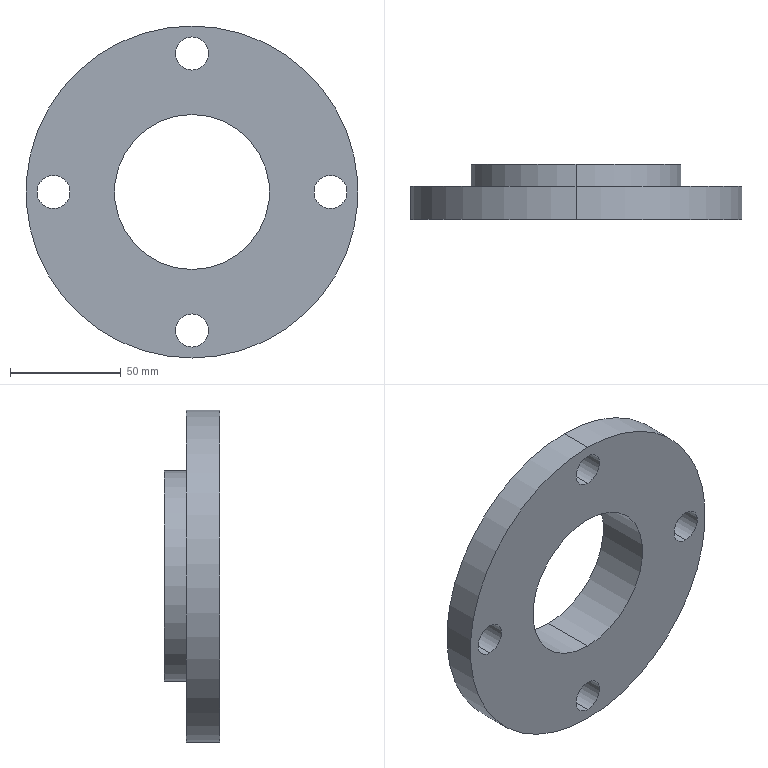Component | SolidWorks | SupportLeg-2 | 1 solid | 17 faces | box 150 x 25 x 150 mm | volume 229140 mm3 | cylinder 14 | plane 3 | commonest cylinder face diameters 15 x8 95 x2 70 x2 150 x2
build123d program:
from build123d import *

# Parameters (mm, degrees)
SKETCH1_R           = 75
SKETCH1_R_2         = 35
SKETCH1_R_3         = 7.5
BOSS_EXTRUDE1_DEPTH = 15
SKETCH2_R           = 47.5
SKETCH2_R_2         = 35
BOSS_EXTRUDE2_DEPTH = 10


with BuildPart() as part:
    # Sketch1 → Boss-Extrude1 (new body)
    with BuildSketch(Plane(origin=(0, 0, 0), x_dir=(1, 0, 0), z_dir=(0, 1, 0))):
        with Locations(Location((0, 0, 0), (0, 0, 270))):
            Circle(SKETCH1_R)
        with Locations(Location((0, 0, 0), (0, 0, 270))):
            Circle(SKETCH1_R_2, mode=Mode.SUBTRACT)
        with Locations(Location((0, 62.566, 0), (0, 0, 270))):
            Circle(SKETCH1_R_3, mode=Mode.SUBTRACT)
        with Locations(Location((62.566, 0, 0), (0, 0, 270))):
            Circle(SKETCH1_R_3, mode=Mode.SUBTRACT)
        with Locations(Location((0, -62.566, 0), (0, 0, 270))):
            Circle(SKETCH1_R_3, mode=Mode.SUBTRACT)
        with Locations(Location((-62.566, 0, 0), (0, 0, 270))):
            Circle(SKETCH1_R_3, mode=Mode.SUBTRACT)
    extrude(amount=BOSS_EXTRUDE1_DEPTH)

    # Sketch2 → Boss-Extrude2 (add)
    with BuildSketch(Plane(origin=(0, 15, 0), x_dir=(1, 0, 0), z_dir=(0, 1, 0))):
        with Locations(Location((0, 0, 0), (0, 0, 270))):
            Circle(SKETCH2_R)
        with Locations(Location((0, 0, 0), (0, 0, 270))):
            Circle(SKETCH2_R_2, mode=Mode.SUBTRACT)
    extrude(amount=BOSS_EXTRUDE2_DEPTH)


solid = part.part

# Placed as in the assembly
solid = solid.moved(Location((-699.263, -180, 149.263), (0, 0, 0)))
STEP:
#1=COLOUR_RGB('',0.7922,0.8196,0.9333);
#2=FILL_AREA_STYLE_COLOUR('',#1);
#3=FILL_AREA_STYLE('',(#2));
#4=SURFACE_STYLE_FILL_AREA(#3);
#5=SURFACE_SIDE_STYLE('',(#4));
#6=SURFACE_STYLE_USAGE(.BOTH.,#5);
#7=PRESENTATION_STYLE_ASSIGNMENT((#6));
#8=CARTESIAN_POINT('',(-27.53,-6.102,7.747));
#9=VERTEX_POINT('',#8);
#10=CARTESIAN_POINT('',(-27.53,-6.102,4.006));
#11=VERTEX_POINT('',#10);
#12=CARTESIAN_POINT('',(-27.53,-6.102,5.877));
#13=DIRECTION('',(0.,1.,0.));
#14=DIRECTION('',(0.,0.,1.));
#15=AXIS2_PLACEMENT_3D('',#12,#13,#14);
#16=CIRCLE('',#15,1.87);
#17=EDGE_CURVE('',#9,#11,#16,.T.);
#18=ORIENTED_EDGE('',*,*,#17,.F.);
#19=CARTESIAN_POINT('',(-27.53,-6.496,7.747));
#20=VERTEX_POINT('',#19);
#21=CARTESIAN_POINT('',(-27.53,-6.102,7.747));
#22=DIRECTION('',(0.,-1.,0.));
#23=VECTOR('',#22,39.37);
#24=LINE('',#21,#23);
#25=EDGE_CURVE('',#9,#20,#24,.T.);
#26=ORIENTED_EDGE('',*,*,#25,.T.);
#27=CARTESIAN_POINT('',(-27.53,-6.496,4.006));
#28=VERTEX_POINT('',#27);
#29=CARTESIAN_POINT('',(-27.53,-6.496,5.877));
#30=DIRECTION('',(0.,1.,0.));
#31=DIRECTION('',(0.,0.,1.));
#32=AXIS2_PLACEMENT_3D('',#29,#30,#31);
#33=CIRCLE('',#32,1.87);
#34=EDGE_CURVE('',#20,#28,#33,.T.);
#35=ORIENTED_EDGE('',*,*,#34,.T.);
#36=CARTESIAN_POINT('',(-27.53,-6.102,4.006));
#37=DIRECTION('',(0.,-1.,0.));
#38=VECTOR('',#37,39.37);
#39=LINE('',#36,#38);
#40=EDGE_CURVE('',#11,#28,#39,.T.);
#41=ORIENTED_EDGE('',*,*,#40,.F.);
#42=EDGE_LOOP('',(#18,#26,#35,#41));
#43=FACE_OUTER_BOUND('',#42,.T.);
#44=CARTESIAN_POINT('',(-27.53,-6.102,5.877));
#45=DIRECTION('',(0.,-1.,0.));
#46=DIRECTION('',(0.,0.,-1.));
#47=AXIS2_PLACEMENT_3D('',#44,#45,#46);
#48=CYLINDRICAL_SURFACE('',#47,1.87);
#49=ADVANCED_FACE('',(#43),#48,.T.);
#50=CARTESIAN_POINT('',(-29.993,-6.496,5.581));
#51=VERTEX_POINT('',#50);
#52=CARTESIAN_POINT('',(-29.993,-6.496,6.172));
#53=VERTEX_POINT('',#52);
#54=CARTESIAN_POINT('',(-29.993,-6.496,5.877));
#55=DIRECTION('',(0.,1.,0.));
#56=DIRECTION('',(0.,0.,1.));
#57=AXIS2_PLACEMENT_3D('',#54,#55,#56);
#58=CIRCLE('',#57,0.2953);
#59=EDGE_CURVE('',#51,#53,#58,.T.);
#60=ORIENTED_EDGE('',*,*,#59,.T.);
#61=CARTESIAN_POINT('',(-29.993,-7.087,6.172));
#62=VERTEX_POINT('',#61);
#63=CARTESIAN_POINT('',(-29.993,-6.496,6.172));
#64=DIRECTION('',(0.,-1.,0.));
#65=VECTOR('',#64,39.37);
#66=LINE('',#63,#65);
#67=EDGE_CURVE('',#53,#62,#66,.T.);
#68=ORIENTED_EDGE('',*,*,#67,.T.);
#69=CARTESIAN_POINT('',(-29.993,-7.087,5.581));
#70=VERTEX_POINT('',#69);
#71=CARTESIAN_POINT('',(-29.993,-7.087,5.877));
#72=DIRECTION('',(0.,1.,0.));
#73=DIRECTION('',(0.,0.,1.));
#74=AXIS2_PLACEMENT_3D('',#71,#72,#73);
#75=CIRCLE('',#74,0.2953);
#76=EDGE_CURVE('',#70,#62,#75,.T.);
#77=ORIENTED_EDGE('',*,*,#76,.F.);
#78=CARTESIAN_POINT('',(-29.993,-6.496,5.581));
#79=DIRECTION('',(0.,-1.,0.));
#80=VECTOR('',#79,39.37);
#81=LINE('',#78,#80);
#82=EDGE_CURVE('',#51,#70,#81,.T.);
#83=ORIENTED_EDGE('',*,*,#82,.F.);
#84=EDGE_LOOP('',(#60,#68,#77,#83));
#85=FACE_OUTER_BOUND('',#84,.T.);
#86=CARTESIAN_POINT('',(-29.993,-6.496,5.877));
#87=DIRECTION('',(0.,-1.,0.));
#88=DIRECTION('',(0.,0.,-1.));
#89=AXIS2_PLACEMENT_3D('',#86,#87,#88);
#90=CYLINDRICAL_SURFACE('',#89,0.2953);
#91=ADVANCED_FACE('',(#85),#90,.F.);
#92=CARTESIAN_POINT('',(-27.53,-6.496,8.044));
#93=VERTEX_POINT('',#92);
#94=CARTESIAN_POINT('',(-27.53,-6.496,8.635));
#95=VERTEX_POINT('',#94);
#96=CARTESIAN_POINT('',(-27.53,-6.496,8.34));
#97=DIRECTION('',(0.,1.,0.));
#98=DIRECTION('',(0.,0.,1.));
#99=AXIS2_PLACEMENT_3D('',#96,#97,#98);
#100=CIRCLE('',#99,0.2953);
#101=EDGE_CURVE('',#93,#95,#100,.T.);
#102=ORIENTED_EDGE('',*,*,#101,.T.);
#103=CARTESIAN_POINT('',(-27.53,-7.087,8.635));
#104=VERTEX_POINT('',#103);
#105=CARTESIAN_POINT('',(-27.53,-6.496,8.635));
#106=DIRECTION('',(0.,-1.,0.));
#107=VECTOR('',#106,39.37);
#108=LINE('',#105,#107);
#109=EDGE_CURVE('',#95,#104,#108,.T.);
#110=ORIENTED_EDGE('',*,*,#109,.T.);
#111=CARTESIAN_POINT('',(-27.53,-7.087,8.044));
#112=VERTEX_POINT('',#111);
#113=CARTESIAN_POINT('',(-27.53,-7.087,8.34));
#114=DIRECTION('',(0.,1.,0.));
#115=DIRECTION('',(0.,0.,1.));
#116=AXIS2_PLACEMENT_3D('',#113,#114,#115);
#117=CIRCLE('',#116,0.2953);
#118=EDGE_CURVE('',#112,#104,#117,.T.);
#119=ORIENTED_EDGE('',*,*,#118,.F.);
#120=CARTESIAN_POINT('',(-27.53,-6.496,8.044));
#121=DIRECTION('',(0.,-1.,0.));
#122=VECTOR('',#121,39.37);
#123=LINE('',#120,#122);
#124=EDGE_CURVE('',#93,#112,#123,.T.);
#125=ORIENTED_EDGE('',*,*,#124,.F.);
#126=EDGE_LOOP('',(#102,#110,#119,#125));
#127=FACE_OUTER_BOUND('',#126,.T.);
#128=CARTESIAN_POINT('',(-27.53,-6.496,8.34));
#129=DIRECTION('',(0.,-1.,0.));
#130=DIRECTION('',(0.,0.,-1.));
#131=AXIS2_PLACEMENT_3D('',#128,#129,#130);
#132=CYLINDRICAL_SURFACE('',#131,0.2953);
#133=ADVANCED_FACE('',(#127),#132,.F.);
#134=CARTESIAN_POINT('',(-25.067,-6.496,5.581));
#135=VERTEX_POINT('',#134);
#136=CARTESIAN_POINT('',(-25.067,-6.496,6.172));
#137=VERTEX_POINT('',#136);
#138=CARTESIAN_POINT('',(-25.067,-6.496,5.877));
#139=DIRECTION('',(0.,1.,0.));
#140=DIRECTION('',(0.,0.,1.));
#141=AXIS2_PLACEMENT_3D('',#138,#139,#140);
#142=CIRCLE('',#141,0.2953);
#143=EDGE_CURVE('',#135,#137,#142,.T.);
#144=ORIENTED_EDGE('',*,*,#143,.T.);
#145=CARTESIAN_POINT('',(-25.067,-7.087,6.172));
#146=VERTEX_POINT('',#145);
#147=CARTESIAN_POINT('',(-25.067,-6.496,6.172));
#148=DIRECTION('',(0.,-1.,0.));
#149=VECTOR('',#148,39.37);
#150=LINE('',#147,#149);
#151=EDGE_CURVE('',#137,#146,#150,.T.);
#152=ORIENTED_EDGE('',*,*,#151,.T.);
#153=CARTESIAN_POINT('',(-25.067,-7.087,5.581));
#154=VERTEX_POINT('',#153);
#155=CARTESIAN_POINT('',(-25.067,-7.087,5.877));
#156=DIRECTION('',(0.,1.,0.));
#157=DIRECTION('',(0.,0.,1.));
#158=AXIS2_PLACEMENT_3D('',#155,#156,#157);
#159=CIRCLE('',#158,0.2953);
#160=EDGE_CURVE('',#154,#146,#159,.T.);
#161=ORIENTED_EDGE('',*,*,#160,.F.);
#162=CARTESIAN_POINT('',(-25.067,-6.496,5.581));
#163=DIRECTION('',(0.,-1.,0.));
#164=VECTOR('',#163,39.37);
#165=LINE('',#162,#164);
#166=EDGE_CURVE('',#135,#154,#165,.T.);
#167=ORIENTED_EDGE('',*,*,#166,.F.);
#168=EDGE_LOOP('',(#144,#152,#161,#167));
#169=FACE_OUTER_BOUND('',#168,.T.);
#170=CARTESIAN_POINT('',(-25.067,-6.496,5.877));
#171=DIRECTION('',(0.,-1.,0.));
#172=DIRECTION('',(0.,0.,-1.));
#173=AXIS2_PLACEMENT_3D('',#170,#171,#172);
#174=CYLINDRICAL_SURFACE('',#173,0.2953);
#175=ADVANCED_FACE('',(#169),#174,.F.);
#176=CARTESIAN_POINT('',(-27.53,-6.496,3.118));
#177=VERTEX_POINT('',#176);
#178=CARTESIAN_POINT('',(-27.53,-6.496,3.709));
#179=VERTEX_POINT('',#178);
#180=CARTESIAN_POINT('',(-27.53,-6.496,3.413));
#181=DIRECTION('',(0.,1.,0.));
#182=DIRECTION('',(0.,0.,1.));
#183=AXIS2_PLACEMENT_3D('',#180,#181,#182);
#184=CIRCLE('',#183,0.2953);
#185=EDGE_CURVE('',#177,#179,#184,.T.);
#186=ORIENTED_EDGE('',*,*,#185,.T.);
#187=CARTESIAN_POINT('',(-27.53,-7.087,3.709));
#188=VERTEX_POINT('',#187);
#189=CARTESIAN_POINT('',(-27.53,-6.496,3.709));
#190=DIRECTION('',(0.,-1.,0.));
#191=VECTOR('',#190,39.37);
#192=LINE('',#189,#191);
#193=EDGE_CURVE('',#179,#188,#192,.T.);
#194=ORIENTED_EDGE('',*,*,#193,.T.);
#195=CARTESIAN_POINT('',(-27.53,-7.087,3.118));
#196=VERTEX_POINT('',#195);
#197=CARTESIAN_POINT('',(-27.53,-7.087,3.413));
#198=DIRECTION('',(0.,1.,0.));
#199=DIRECTION('',(0.,0.,1.));
#200=AXIS2_PLACEMENT_3D('',#197,#198,#199);
#201=CIRCLE('',#200,0.2953);
#202=EDGE_CURVE('',#196,#188,#201,.T.);
#203=ORIENTED_EDGE('',*,*,#202,.F.);
#204=CARTESIAN_POINT('',(-27.53,-6.496,3.118));
#205=DIRECTION('',(0.,-1.,0.));
#206=VECTOR('',#205,39.37);
#207=LINE('',#204,#206);
#208=EDGE_CURVE('',#177,#196,#207,.T.);
#209=ORIENTED_EDGE('',*,*,#208,.F.);
#210=EDGE_LOOP('',(#186,#194,#203,#209));
#211=FACE_OUTER_BOUND('',#210,.T.);
#212=CARTESIAN_POINT('',(-27.53,-6.496,3.413));
#213=DIRECTION('',(0.,-1.,0.));
#214=DIRECTION('',(0.,0.,-1.));
#215=AXIS2_PLACEMENT_3D('',#212,#213,#214);
#216=CYLINDRICAL_SURFACE('',#215,0.2953);
#217=ADVANCED_FACE('',(#211),#216,.F.);
#218=CARTESIAN_POINT('',(-27.53,-6.102,4.499));
#219=VERTEX_POINT('',#218);
#220=CARTESIAN_POINT('',(-27.53,-6.102,7.254));
#221=VERTEX_POINT('',#220);
#222=CARTESIAN_POINT('',(-27.53,-6.102,5.877));
#223=DIRECTION('',(0.,1.,0.));
#224=DIRECTION('',(0.,0.,1.));
#225=AXIS2_PLACEMENT_3D('',#222,#223,#224);
#226=CIRCLE('',#225,1.378);
#227=EDGE_CURVE('',#219,#221,#226,.T.);
#228=ORIENTED_EDGE('',*,*,#227,.T.);
#229=CARTESIAN_POINT('',(-27.53,-7.087,7.254));
#230=VERTEX_POINT('',#229);
#231=CARTESIAN_POINT('',(-27.53,-6.496,7.254));
#232=DIRECTION('',(0.,-1.,0.));
#233=VECTOR('',#232,39.37);
#234=LINE('',#231,#233);
#235=EDGE_CURVE('',#221,#230,#234,.T.);
#236=ORIENTED_EDGE('',*,*,#235,.T.);
#237=CARTESIAN_POINT('',(-27.53,-7.087,4.499));
#238=VERTEX_POINT('',#237);
#239=CARTESIAN_POINT('',(-27.53,-7.087,5.877));
#240=DIRECTION('',(0.,1.,0.));
#241=DIRECTION('',(0.,0.,1.));
#242=AXIS2_PLACEMENT_3D('',#239,#240,#241);
#243=CIRCLE('',#242,1.378);
#244=EDGE_CURVE('',#238,#230,#243,.T.);
#245=ORIENTED_EDGE('',*,*,#244,.F.);
#246=CARTESIAN_POINT('',(-27.53,-6.496,4.499));
#247=DIRECTION('',(0.,-1.,0.));
#248=VECTOR('',#247,39.37);
#249=LINE('',#246,#248);
#250=EDGE_CURVE('',#219,#238,#249,.T.);
#251=ORIENTED_EDGE('',*,*,#250,.F.);
#252=EDGE_LOOP('',(#228,#236,#245,#251));
#253=FACE_OUTER_BOUND('',#252,.T.);
#254=CARTESIAN_POINT('',(-27.53,-6.496,5.877));
#255=DIRECTION('',(0.,-1.,0.));
#256=DIRECTION('',(0.,0.,-1.));
#257=AXIS2_PLACEMENT_3D('',#254,#255,#256);
#258=CYLINDRICAL_SURFACE('',#257,1.378);
#259=ADVANCED_FACE('',(#253),#258,.F.);
#260=CARTESIAN_POINT('',(-27.53,-6.496,8.829));
#261=VERTEX_POINT('',#260);
#262=CARTESIAN_POINT('',(-27.53,-6.496,2.924));
#263=VERTEX_POINT('',#262);
#264=CARTESIAN_POINT('',(-27.53,-6.496,5.877));
#265=DIRECTION('',(0.,1.,0.));
#266=DIRECTION('',(0.,0.,1.));
#267=AXIS2_PLACEMENT_3D('',#264,#265,#266);
#268=CIRCLE('',#267,2.953);
#269=EDGE_CURVE('',#261,#263,#268,.T.);
#270=ORIENTED_EDGE('',*,*,#269,.F.);
#271=CARTESIAN_POINT('',(-27.53,-7.087,8.829));
#272=VERTEX_POINT('',#271);
#273=CARTESIAN_POINT('',(-27.53,-6.496,8.829));
#274=DIRECTION('',(0.,-1.,0.));
#275=VECTOR('',#274,39.37);
#276=LINE('',#273,#275);
#277=EDGE_CURVE('',#261,#272,#276,.T.);
#278=ORIENTED_EDGE('',*,*,#277,.T.);
#279=CARTESIAN_POINT('',(-27.53,-7.087,2.924));
#280=VERTEX_POINT('',#279);
#281=CARTESIAN_POINT('',(-27.53,-7.087,5.877));
#282=DIRECTION('',(0.,1.,0.));
#283=DIRECTION('',(0.,0.,1.));
#284=AXIS2_PLACEMENT_3D('',#281,#282,#283);
#285=CIRCLE('',#284,2.953);
#286=EDGE_CURVE('',#272,#280,#285,.T.);
#287=ORIENTED_EDGE('',*,*,#286,.T.);
#288=CARTESIAN_POINT('',(-27.53,-6.496,2.924));
#289=DIRECTION('',(0.,-1.,0.));
#290=VECTOR('',#289,39.37);
#291=LINE('',#288,#290);
#292=EDGE_CURVE('',#263,#280,#291,.T.);
#293=ORIENTED_EDGE('',*,*,#292,.F.);
#294=EDGE_LOOP('',(#270,#278,#287,#293));
#295=FACE_OUTER_BOUND('',#294,.T.);
#296=CARTESIAN_POINT('',(-27.53,-6.496,5.877));
#297=DIRECTION('',(0.,-1.,0.));
#298=DIRECTION('',(0.,0.,-1.));
#299=AXIS2_PLACEMENT_3D('',#296,#297,#298);
#300=CYLINDRICAL_SURFACE('',#299,2.953);
#301=ADVANCED_FACE('',(#295),#300,.T.);
#302=CARTESIAN_POINT('',(-27.53,-6.496,5.877));
#303=DIRECTION('',(0.,1.,0.));
#304=DIRECTION('',(0.,0.,1.));
#305=AXIS2_PLACEMENT_3D('',#302,#303,#304);
#306=CIRCLE('',#305,1.87);
#307=EDGE_CURVE('',#28,#20,#306,.T.);
#308=ORIENTED_EDGE('',*,*,#307,.F.);
#309=ORIENTED_EDGE('',*,*,#34,.F.);
#310=EDGE_LOOP('',(#308,#309));
#311=FACE_BOUND('',#310,.T.);
#312=ORIENTED_EDGE('',*,*,#101,.F.);
#313=CARTESIAN_POINT('',(-27.53,-6.496,8.34));
#314=DIRECTION('',(0.,1.,0.));
#315=DIRECTION('',(0.,0.,1.));
#316=AXIS2_PLACEMENT_3D('',#313,#314,#315);
#317=CIRCLE('',#316,0.2953);
#318=EDGE_CURVE('',#95,#93,#317,.T.);
#319=ORIENTED_EDGE('',*,*,#318,.F.);
#320=EDGE_LOOP('',(#312,#319));
#321=FACE_BOUND('',#320,.T.);
#322=ORIENTED_EDGE('',*,*,#185,.F.);
#323=CARTESIAN_POINT('',(-27.53,-6.496,3.413));
#324=DIRECTION('',(0.,1.,0.));
#325=DIRECTION('',(0.,0.,1.));
#326=AXIS2_PLACEMENT_3D('',#323,#324,#325);
#327=CIRCLE('',#326,0.2953);
#328=EDGE_CURVE('',#179,#177,#327,.T.);
#329=ORIENTED_EDGE('',*,*,#328,.F.);
#330=EDGE_LOOP('',(#322,#329));
#331=FACE_BOUND('',#330,.T.);
#332=CARTESIAN_POINT('',(-27.53,-6.496,5.877));
#333=DIRECTION('',(0.,1.,0.));
#334=DIRECTION('',(0.,0.,1.));
#335=AXIS2_PLACEMENT_3D('',#332,#333,#334);
#336=CIRCLE('',#335,2.953);
#337=EDGE_CURVE('',#263,#261,#336,.T.);
#338=ORIENTED_EDGE('',*,*,#337,.T.);
#339=ORIENTED_EDGE('',*,*,#269,.T.);
#340=EDGE_LOOP('',(#338,#339));
#341=FACE_OUTER_BOUND('',#340,.T.);
#342=ORIENTED_EDGE('',*,*,#143,.F.);
#343=CARTESIAN_POINT('',(-25.067,-6.496,5.877));
#344=DIRECTION('',(0.,1.,0.));
#345=DIRECTION('',(0.,0.,1.));
#346=AXIS2_PLACEMENT_3D('',#343,#344,#345);
#347=CIRCLE('',#346,0.2953);
#348=EDGE_CURVE('',#137,#135,#347,.T.);
#349=ORIENTED_EDGE('',*,*,#348,.F.);
#350=EDGE_LOOP('',(#342,#349));
#351=FACE_BOUND('',#350,.T.);
#352=ORIENTED_EDGE('',*,*,#59,.F.);
#353=CARTESIAN_POINT('',(-29.993,-6.496,5.877));
#354=DIRECTION('',(0.,1.,0.));
#355=DIRECTION('',(0.,0.,1.));
#356=AXIS2_PLACEMENT_3D('',#353,#354,#355);
#357=CIRCLE('',#356,0.2953);
#358=EDGE_CURVE('',#53,#51,#357,.T.);
#359=ORIENTED_EDGE('',*,*,#358,.F.);
#360=EDGE_LOOP('',(#352,#359));
#361=FACE_BOUND('',#360,.T.);
#362=CARTESIAN_POINT('',(-27.53,-6.496,5.877));
#363=DIRECTION('',(0.,1.,0.));
#364=DIRECTION('',(0.,0.,1.));
#365=AXIS2_PLACEMENT_3D('',#362,#363,#364);
#366=PLANE('',#365);
#367=ADVANCED_FACE('',(#311,#321,#331,#341,#351,#361),#366,.T.);
#368=CARTESIAN_POINT('',(-27.53,-7.087,5.877));
#369=DIRECTION('',(0.,1.,0.));
#370=DIRECTION('',(0.,0.,1.));
#371=AXIS2_PLACEMENT_3D('',#368,#369,#370);
#372=CIRCLE('',#371,2.953);
#373=EDGE_CURVE('',#280,#272,#372,.T.);
#374=ORIENTED_EDGE('',*,*,#373,.F.);
#375=ORIENTED_EDGE('',*,*,#286,.F.);
#376=EDGE_LOOP('',(#374,#375));
#377=FACE_OUTER_BOUND('',#376,.T.);
#378=ORIENTED_EDGE('',*,*,#244,.T.);
#379=CARTESIAN_POINT('',(-27.53,-7.087,5.877));
#380=DIRECTION('',(0.,1.,0.));
#381=DIRECTION('',(0.,0.,1.));
#382=AXIS2_PLACEMENT_3D('',#379,#380,#381);
#383=CIRCLE('',#382,1.378);
#384=EDGE_CURVE('',#230,#238,#383,.T.);
#385=ORIENTED_EDGE('',*,*,#384,.T.);
#386=EDGE_LOOP('',(#378,#385));
#387=FACE_BOUND('',#386,.T.);
#388=ORIENTED_EDGE('',*,*,#202,.T.);
#389=CARTESIAN_POINT('',(-27.53,-7.087,3.413));
#390=DIRECTION('',(0.,1.,0.));
#391=DIRECTION('',(0.,0.,1.));
#392=AXIS2_PLACEMENT_3D('',#389,#390,#391);
#393=CIRCLE('',#392,0.2953);
#394=EDGE_CURVE('',#188,#196,#393,.T.);
#395=ORIENTED_EDGE('',*,*,#394,.T.);
#396=EDGE_LOOP('',(#388,#395));
#397=FACE_BOUND('',#396,.T.);
#398=ORIENTED_EDGE('',*,*,#160,.T.);
#399=CARTESIAN_POINT('',(-25.067,-7.087,5.877));
#400=DIRECTION('',(0.,1.,0.));
#401=DIRECTION('',(0.,0.,1.));
#402=AXIS2_PLACEMENT_3D('',#399,#400,#401);
#403=CIRCLE('',#402,0.2953);
#404=EDGE_CURVE('',#146,#154,#403,.T.);
#405=ORIENTED_EDGE('',*,*,#404,.T.);
#406=EDGE_LOOP('',(#398,#405));
#407=FACE_BOUND('',#406,.T.);
#408=ORIENTED_EDGE('',*,*,#118,.T.);
#409=CARTESIAN_POINT('',(-27.53,-7.087,8.34));
#410=DIRECTION('',(0.,1.,0.));
#411=DIRECTION('',(0.,0.,1.));
#412=AXIS2_PLACEMENT_3D('',#409,#410,#411);
#413=CIRCLE('',#412,0.2953);
#414=EDGE_CURVE('',#104,#112,#413,.T.);
#415=ORIENTED_EDGE('',*,*,#414,.T.);
#416=EDGE_LOOP('',(#408,#415));
#417=FACE_BOUND('',#416,.T.);
#418=ORIENTED_EDGE('',*,*,#76,.T.);
#419=CARTESIAN_POINT('',(-29.993,-7.087,5.877));
#420=DIRECTION('',(0.,1.,0.));
#421=DIRECTION('',(0.,0.,1.));
#422=AXIS2_PLACEMENT_3D('',#419,#420,#421);
#423=CIRCLE('',#422,0.2953);
#424=EDGE_CURVE('',#62,#70,#423,.T.);
#425=ORIENTED_EDGE('',*,*,#424,.T.);
#426=EDGE_LOOP('',(#418,#425));
#427=FACE_BOUND('',#426,.T.);
#428=CARTESIAN_POINT('',(-27.53,-7.087,5.877));
#429=DIRECTION('',(0.,1.,0.));
#430=DIRECTION('',(0.,0.,1.));
#431=AXIS2_PLACEMENT_3D('',#428,#429,#430);
#432=PLANE('',#431);
#433=ADVANCED_FACE('',(#377,#387,#397,#407,#417,#427),#432,.F.);
#434=ORIENTED_EDGE('',*,*,#277,.F.);
#435=ORIENTED_EDGE('',*,*,#337,.F.);
#436=ORIENTED_EDGE('',*,*,#292,.T.);
#437=ORIENTED_EDGE('',*,*,#373,.T.);
#438=EDGE_LOOP('',(#434,#435,#436,#437));
#439=FACE_OUTER_BOUND('',#438,.T.);
#440=CARTESIAN_POINT('',(-27.53,-6.496,5.877));
#441=DIRECTION('',(0.,-1.,0.));
#442=DIRECTION('',(0.,0.,-1.));
#443=AXIS2_PLACEMENT_3D('',#440,#441,#442);
#444=CYLINDRICAL_SURFACE('',#443,2.953);
#445=ADVANCED_FACE('',(#439),#444,.T.);
#446=ORIENTED_EDGE('',*,*,#235,.F.);
#447=CARTESIAN_POINT('',(-27.53,-6.102,5.877));
#448=DIRECTION('',(0.,1.,0.));
#449=DIRECTION('',(0.,0.,1.));
#450=AXIS2_PLACEMENT_3D('',#447,#448,#449);
#451=CIRCLE('',#450,1.378);
#452=EDGE_CURVE('',#221,#219,#451,.T.);
#453=ORIENTED_EDGE('',*,*,#452,.T.);
#454=ORIENTED_EDGE('',*,*,#250,.T.);
#455=ORIENTED_EDGE('',*,*,#384,.F.);
#456=EDGE_LOOP('',(#446,#453,#454,#455));
#457=FACE_OUTER_BOUND('',#456,.T.);
#458=CARTESIAN_POINT('',(-27.53,-6.496,5.877));
#459=DIRECTION('',(0.,-1.,0.));
#460=DIRECTION('',(0.,0.,-1.));
#461=AXIS2_PLACEMENT_3D('',#458,#459,#460);
#462=CYLINDRICAL_SURFACE('',#461,1.378);
#463=ADVANCED_FACE('',(#457),#462,.F.);
#464=ORIENTED_EDGE('',*,*,#193,.F.);
#465=ORIENTED_EDGE('',*,*,#328,.T.);
#466=ORIENTED_EDGE('',*,*,#208,.T.);
#467=ORIENTED_EDGE('',*,*,#394,.F.);
#468=EDGE_LOOP('',(#464,#465,#466,#467));
#469=FACE_OUTER_BOUND('',#468,.T.);
#470=CARTESIAN_POINT('',(-27.53,-6.496,3.413));
#471=DIRECTION('',(0.,-1.,0.));
#472=DIRECTION('',(0.,0.,-1.));
#473=AXIS2_PLACEMENT_3D('',#470,#471,#472);
#474=CYLINDRICAL_SURFACE('',#473,0.2953);
#475=ADVANCED_FACE('',(#469),#474,.F.);
#476=ORIENTED_EDGE('',*,*,#151,.F.);
#477=ORIENTED_EDGE('',*,*,#348,.T.);
#478=ORIENTED_EDGE('',*,*,#166,.T.);
#479=ORIENTED_EDGE('',*,*,#404,.F.);
#480=EDGE_LOOP('',(#476,#477,#478,#479));
#481=FACE_OUTER_BOUND('',#480,.T.);
#482=CARTESIAN_POINT('',(-25.067,-6.496,5.877));
#483=DIRECTION('',(0.,-1.,0.));
#484=DIRECTION('',(0.,0.,-1.));
#485=AXIS2_PLACEMENT_3D('',#482,#483,#484);
#486=CYLINDRICAL_SURFACE('',#485,0.2953);
#487=ADVANCED_FACE('',(#481),#486,.F.);
#488=ORIENTED_EDGE('',*,*,#109,.F.);
#489=ORIENTED_EDGE('',*,*,#318,.T.);
#490=ORIENTED_EDGE('',*,*,#124,.T.);
#491=ORIENTED_EDGE('',*,*,#414,.F.);
#492=EDGE_LOOP('',(#488,#489,#490,#491));
#493=FACE_OUTER_BOUND('',#492,.T.);
#494=CARTESIAN_POINT('',(-27.53,-6.496,8.34));
#495=DIRECTION('',(0.,-1.,0.));
#496=DIRECTION('',(0.,0.,-1.));
#497=AXIS2_PLACEMENT_3D('',#494,#495,#496);
#498=CYLINDRICAL_SURFACE('',#497,0.2953);
#499=ADVANCED_FACE('',(#493),#498,.F.);
#500=ORIENTED_EDGE('',*,*,#67,.F.);
#501=ORIENTED_EDGE('',*,*,#358,.T.);
#502=ORIENTED_EDGE('',*,*,#82,.T.);
#503=ORIENTED_EDGE('',*,*,#424,.F.);
#504=EDGE_LOOP('',(#500,#501,#502,#503));
#505=FACE_OUTER_BOUND('',#504,.T.);
#506=CARTESIAN_POINT('',(-29.993,-6.496,5.877));
#507=DIRECTION('',(0.,-1.,0.));
#508=DIRECTION('',(0.,0.,-1.));
#509=AXIS2_PLACEMENT_3D('',#506,#507,#508);
#510=CYLINDRICAL_SURFACE('',#509,0.2953);
#511=ADVANCED_FACE('',(#505),#510,.F.);
#512=CARTESIAN_POINT('',(-27.53,-6.102,5.877));
#513=DIRECTION('',(0.,1.,0.));
#514=DIRECTION('',(0.,0.,1.));
#515=AXIS2_PLACEMENT_3D('',#512,#513,#514);
#516=CIRCLE('',#515,1.87);
#517=EDGE_CURVE('',#11,#9,#516,.T.);
#518=ORIENTED_EDGE('',*,*,#517,.T.);
#519=ORIENTED_EDGE('',*,*,#17,.T.);
#520=EDGE_LOOP('',(#518,#519));
#521=FACE_OUTER_BOUND('',#520,.T.);
#522=ORIENTED_EDGE('',*,*,#227,.F.);
#523=ORIENTED_EDGE('',*,*,#452,.F.);
#524=EDGE_LOOP('',(#522,#523));
#525=FACE_BOUND('',#524,.T.);
#526=CARTESIAN_POINT('',(-27.53,-6.102,5.877));
#527=DIRECTION('',(0.,1.,0.));
#528=DIRECTION('',(0.,0.,1.));
#529=AXIS2_PLACEMENT_3D('',#526,#527,#528);
#530=PLANE('',#529);
#531=ADVANCED_FACE('',(#521,#525),#530,.T.);
#532=ORIENTED_EDGE('',*,*,#25,.F.);
#533=ORIENTED_EDGE('',*,*,#517,.F.);
#534=ORIENTED_EDGE('',*,*,#40,.T.);
#535=ORIENTED_EDGE('',*,*,#307,.T.);
#536=EDGE_LOOP('',(#532,#533,#534,#535));
#537=FACE_OUTER_BOUND('',#536,.T.);
#538=CARTESIAN_POINT('',(-27.53,-6.102,5.877));
#539=DIRECTION('',(0.,-1.,0.));
#540=DIRECTION('',(0.,0.,-1.));
#541=AXIS2_PLACEMENT_3D('',#538,#539,#540);
#542=CYLINDRICAL_SURFACE('',#541,1.87);
#543=ADVANCED_FACE('',(#537),#542,.T.);
#544=CLOSED_SHELL('',(#49,#91,#133,#175,#217,#259,#301,#367,#433,#445,#463,#475,#487,#499,#511,#531,#543));
#545=MANIFOLD_SOLID_BREP('',#544);
#546=STYLED_ITEM('',(#7),#545);
#547=(LENGTH_UNIT()NAMED_UNIT(*)SI_UNIT($,.METRE.));
#548=LENGTH_MEASURE_WITH_UNIT(LENGTH_MEASURE(0.0254),#547);
#549=DIMENSIONAL_EXPONENTS(1.,0.,0.,0.,0.,0.,0.);
#550=(CONVERSION_BASED_UNIT('',#548)LENGTH_UNIT()NAMED_UNIT(#549));
#551=UNCERTAINTY_MEASURE_WITH_UNIT(LENGTH_MEASURE(0.00001),#550,'','');
#552=(NAMED_UNIT(*)PLANE_ANGLE_UNIT()SI_UNIT($,.RADIAN.));
#553=(NAMED_UNIT(*)SI_UNIT($,.STERADIAN.)SOLID_ANGLE_UNIT());
#554=(GEOMETRIC_REPRESENTATION_CONTEXT(3)GLOBAL_UNCERTAINTY_ASSIGNED_CONTEXT((#551))GLOBAL_UNIT_ASSIGNED_CONTEXT((#550,#552,#553))REPRESENTATION_CONTEXT('',''));
#555=MECHANICAL_DESIGN_GEOMETRIC_PRESENTATION_REPRESENTATION('',(#546),#554);
#556=CARTESIAN_POINT('',(0.,0.,0.));
#557=DIRECTION('',(0.,0.,1.));
#558=DIRECTION('',(1.,0.,0.));
#559=AXIS2_PLACEMENT_3D('',#556,#557,#558);
#560=(LENGTH_UNIT()NAMED_UNIT(*)SI_UNIT($,.METRE.));
#561=LENGTH_MEASURE_WITH_UNIT(LENGTH_MEASURE(0.0254),#560);
#562=DIMENSIONAL_EXPONENTS(1.,0.,0.,0.,0.,0.,0.);
#563=(CONVERSION_BASED_UNIT('',#561)LENGTH_UNIT()NAMED_UNIT(#562));
#564=UNCERTAINTY_MEASURE_WITH_UNIT(LENGTH_MEASURE(0.00001),#563,'','');
#565=(NAMED_UNIT(*)PLANE_ANGLE_UNIT()SI_UNIT($,.RADIAN.));
#566=(NAMED_UNIT(*)SI_UNIT($,.STERADIAN.)SOLID_ANGLE_UNIT());
#567=(GEOMETRIC_REPRESENTATION_CONTEXT(3)GLOBAL_UNCERTAINTY_ASSIGNED_CONTEXT((#564))GLOBAL_UNIT_ASSIGNED_CONTEXT((#563,#565,#566))REPRESENTATION_CONTEXT('',''));
#568=ADVANCED_BREP_SHAPE_REPRESENTATION('',(#545,#559),#567);
#569=PRESENTATION_LAYER_ASSIGNMENT('','',(#546));